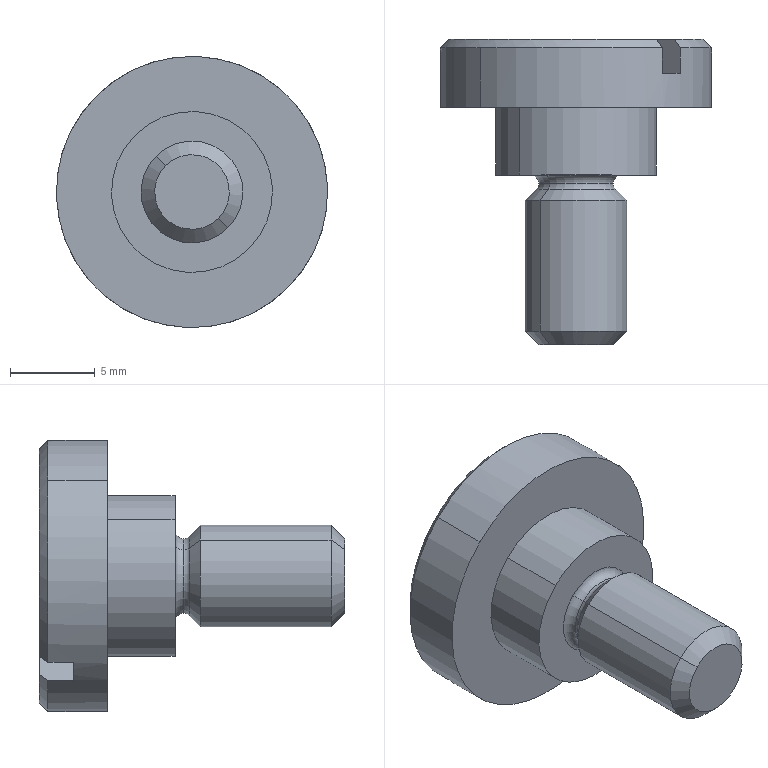Component | SolidWorks | JB_T8045.5-1999DrillBushingScrewM6-1 | 1 solid | 25 faces | box 16 x 18 x 16 mm | volume 1298 mm3 | plane 8 | cone 7 | cylinder 6 | torus 4 | commonest cylinder face diameters 6 x2 9.5 x2 16 x2 | material Nickel
STEP:
#1=COLOUR_RGB('',0.7922,0.8196,0.9333);
#2=FILL_AREA_STYLE_COLOUR('',#1);
#3=FILL_AREA_STYLE('',(#2));
#4=SURFACE_STYLE_FILL_AREA(#3);
#5=SURFACE_SIDE_STYLE('',(#4));
#6=SURFACE_STYLE_USAGE(.BOTH.,#5);
#7=PRESENTATION_STYLE_ASSIGNMENT((#6));
#8=CARTESIAN_POINT('',(0.06125,11.575,1.415));
#9=VERTEX_POINT('',#8);
#10=CARTESIAN_POINT('',(-0.06125,11.575,1.538));
#11=VERTEX_POINT('',#10);
#12=CARTESIAN_POINT('',(0.,11.575,1.476));
#13=DIRECTION('',(0.,-1.,0.));
#14=DIRECTION('',(0.7071,0.,-0.7071));
#15=AXIS2_PLACEMENT_3D('',#12,#13,#14);
#16=CIRCLE('',#15,0.08661);
#17=EDGE_CURVE('',#9,#11,#16,.T.);
#18=ORIENTED_EDGE('',*,*,#17,.F.);
#19=CARTESIAN_POINT('',(0.08352,11.606,1.393));
#20=VERTEX_POINT('',#19);
#21=CARTESIAN_POINT('',(0.06125,11.575,1.415));
#22=DIRECTION('',(0.5,0.7071,-0.5));
#23=VECTOR('',#22,39.37);
#24=LINE('',#21,#23);
#25=EDGE_CURVE('',#9,#20,#24,.T.);
#26=ORIENTED_EDGE('',*,*,#25,.T.);
#27=CARTESIAN_POINT('',(-0.08352,11.606,1.56));
#28=VERTEX_POINT('',#27);
#29=CARTESIAN_POINT('',(0.,11.606,1.476));
#30=DIRECTION('',(0.,1.,0.));
#31=DIRECTION('',(0.7071,0.,-0.7071));
#32=AXIS2_PLACEMENT_3D('',#29,#30,#31);
#33=CIRCLE('',#32,0.1181);
#34=EDGE_CURVE('',#28,#20,#33,.T.);
#35=ORIENTED_EDGE('',*,*,#34,.F.);
#36=CARTESIAN_POINT('',(-0.06125,11.575,1.538));
#37=DIRECTION('',(-0.5,0.7071,0.5));
#38=VECTOR('',#37,39.37);
#39=LINE('',#36,#38);
#40=EDGE_CURVE('',#11,#28,#39,.T.);
#41=ORIENTED_EDGE('',*,*,#40,.F.);
#42=EDGE_LOOP('',(#18,#26,#35,#41));
#43=FACE_OUTER_BOUND('',#42,.T.);
#44=CARTESIAN_POINT('',(0.,11.575,1.476));
#45=DIRECTION('',(0.,1.,0.));
#46=DIRECTION('',(-0.7071,0.,0.7071));
#47=AXIS2_PLACEMENT_3D('',#44,#45,#46);
#48=CONICAL_SURFACE('',#47,0.08661,0.7854);
#49=ADVANCED_FACE('',(#43),#48,.T.);
#50=CARTESIAN_POINT('',(0.06125,11.949,1.415));
#51=VERTEX_POINT('',#50);
#52=CARTESIAN_POINT('',(-0.06125,11.949,1.538));
#53=VERTEX_POINT('',#52);
#54=CARTESIAN_POINT('',(0.,11.949,1.476));
#55=DIRECTION('',(0.,1.,0.));
#56=DIRECTION('',(0.7071,0.,-0.7071));
#57=AXIS2_PLACEMENT_3D('',#54,#55,#56);
#58=CIRCLE('',#57,0.08661);
#59=EDGE_CURVE('',#51,#53,#58,.T.);
#60=ORIENTED_EDGE('',*,*,#59,.T.);
#61=CARTESIAN_POINT('',(-0.07516,11.969,1.552));
#62=VERTEX_POINT('',#61);
#63=CARTESIAN_POINT('',(-0.07516,11.949,1.552));
#64=DIRECTION('',(0.7071,0.,0.7071));
#65=DIRECTION('',(0.7071,0.,-0.7071));
#66=AXIS2_PLACEMENT_3D('',#63,#64,#65);
#67=CIRCLE('',#66,0.01969);
#68=EDGE_CURVE('',#53,#62,#67,.T.);
#69=ORIENTED_EDGE('',*,*,#68,.T.);
#70=CARTESIAN_POINT('',(0.07516,11.969,1.401));
#71=VERTEX_POINT('',#70);
#72=CARTESIAN_POINT('',(0.,11.969,1.476));
#73=DIRECTION('',(0.,1.,0.));
#74=DIRECTION('',(0.7071,0.,-0.7071));
#75=AXIS2_PLACEMENT_3D('',#72,#73,#74);
#76=CIRCLE('',#75,0.1063);
#77=EDGE_CURVE('',#71,#62,#76,.T.);
#78=ORIENTED_EDGE('',*,*,#77,.F.);
#79=CARTESIAN_POINT('',(0.07516,11.949,1.401));
#80=DIRECTION('',(-0.7071,0.,-0.7071));
#81=DIRECTION('',(-0.7071,0.,0.7071));
#82=AXIS2_PLACEMENT_3D('',#79,#80,#81);
#83=CIRCLE('',#82,0.01969);
#84=EDGE_CURVE('',#51,#71,#83,.T.);
#85=ORIENTED_EDGE('',*,*,#84,.F.);
#86=EDGE_LOOP('',(#60,#69,#78,#85));
#87=FACE_OUTER_BOUND('',#86,.T.);
#88=CARTESIAN_POINT('',(0.,11.949,1.476));
#89=DIRECTION('',(0.,-1.,0.));
#90=DIRECTION('',(0.7071,0.,-0.7071));
#91=AXIS2_PLACEMENT_3D('',#88,#89,#90);
#92=TOROIDAL_SURFACE('',#91,0.1063,0.01969);
#93=ADVANCED_FACE('',(#87),#92,.F.);
#94=CARTESIAN_POINT('',(-0.06532,11.935,1.542));
#95=VERTEX_POINT('',#94);
#96=CARTESIAN_POINT('',(0.06532,11.935,1.411));
#97=VERTEX_POINT('',#96);
#98=CARTESIAN_POINT('',(0.,11.935,1.476));
#99=DIRECTION('',(0.,-1.,0.));
#100=DIRECTION('',(-0.7071,0.,0.7071));
#101=AXIS2_PLACEMENT_3D('',#98,#99,#100);
#102=CIRCLE('',#101,0.09238);
#103=EDGE_CURVE('',#95,#97,#102,.T.);
#104=ORIENTED_EDGE('',*,*,#103,.F.);
#105=CARTESIAN_POINT('',(-0.07516,11.949,1.552));
#106=DIRECTION('',(0.7071,0.,0.7071));
#107=DIRECTION('',(0.7071,0.,-0.7071));
#108=AXIS2_PLACEMENT_3D('',#105,#106,#107);
#109=CIRCLE('',#108,0.01969);
#110=EDGE_CURVE('',#95,#53,#109,.T.);
#111=ORIENTED_EDGE('',*,*,#110,.T.);
#112=ORIENTED_EDGE('',*,*,#59,.F.);
#113=CARTESIAN_POINT('',(0.07516,11.949,1.401));
#114=DIRECTION('',(-0.7071,0.,-0.7071));
#115=DIRECTION('',(-0.7071,0.,0.7071));
#116=AXIS2_PLACEMENT_3D('',#113,#114,#115);
#117=CIRCLE('',#116,0.01969);
#118=EDGE_CURVE('',#97,#51,#117,.T.);
#119=ORIENTED_EDGE('',*,*,#118,.F.);
#120=EDGE_LOOP('',(#104,#111,#112,#119));
#121=FACE_OUTER_BOUND('',#120,.T.);
#122=CARTESIAN_POINT('',(0.,11.949,1.476));
#123=DIRECTION('',(0.,-1.,0.));
#124=DIRECTION('',(0.7071,0.,-0.7071));
#125=AXIS2_PLACEMENT_3D('',#122,#123,#124);
#126=TOROIDAL_SURFACE('',#125,0.1063,0.01969);
#127=ADVANCED_FACE('',(#121),#126,.F.);
#128=CARTESIAN_POINT('',(0.,11.935,1.476));
#129=DIRECTION('',(0.,-1.,0.));
#130=DIRECTION('',(-0.7071,0.,0.7071));
#131=AXIS2_PLACEMENT_3D('',#128,#129,#130);
#132=CIRCLE('',#131,0.09238);
#133=EDGE_CURVE('',#97,#95,#132,.T.);
#134=ORIENTED_EDGE('',*,*,#133,.T.);
#135=CARTESIAN_POINT('',(-0.08352,11.909,1.56));
#136=VERTEX_POINT('',#135);
#137=CARTESIAN_POINT('',(-0.08352,11.909,1.56));
#138=DIRECTION('',(-0.5,-0.7071,0.5));
#139=VECTOR('',#138,39.37);
#140=LINE('',#137,#139);
#141=EDGE_CURVE('',#95,#136,#140,.T.);
#142=ORIENTED_EDGE('',*,*,#141,.T.);
#143=CARTESIAN_POINT('',(0.08352,11.909,1.393));
#144=VERTEX_POINT('',#143);
#145=CARTESIAN_POINT('',(0.,11.909,1.476));
#146=DIRECTION('',(0.,-1.,0.));
#147=DIRECTION('',(0.7071,0.,-0.7071));
#148=AXIS2_PLACEMENT_3D('',#145,#146,#147);
#149=CIRCLE('',#148,0.1181);
#150=EDGE_CURVE('',#144,#136,#149,.T.);
#151=ORIENTED_EDGE('',*,*,#150,.F.);
#152=CARTESIAN_POINT('',(0.08352,11.909,1.393));
#153=DIRECTION('',(0.5,-0.7071,-0.5));
#154=VECTOR('',#153,39.37);
#155=LINE('',#152,#154);
#156=EDGE_CURVE('',#97,#144,#155,.T.);
#157=ORIENTED_EDGE('',*,*,#156,.F.);
#158=EDGE_LOOP('',(#134,#142,#151,#157));
#159=FACE_OUTER_BOUND('',#158,.T.);
#160=CARTESIAN_POINT('',(0.,11.909,1.476));
#161=DIRECTION('',(0.,-1.,0.));
#162=DIRECTION('',(0.7071,0.,-0.7071));
#163=AXIS2_PLACEMENT_3D('',#160,#161,#162);
#164=CONICAL_SURFACE('',#163,0.1181,0.7854);
#165=ADVANCED_FACE('',(#159),#164,.T.);
#166=ORIENTED_EDGE('',*,*,#34,.T.);
#167=CARTESIAN_POINT('',(0.08352,11.575,1.393));
#168=DIRECTION('',(0.,1.,0.));
#169=VECTOR('',#168,39.37);
#170=LINE('',#167,#169);
#171=EDGE_CURVE('',#20,#144,#170,.T.);
#172=ORIENTED_EDGE('',*,*,#171,.T.);
#173=ORIENTED_EDGE('',*,*,#150,.T.);
#174=CARTESIAN_POINT('',(-0.08352,11.575,1.56));
#175=DIRECTION('',(0.,1.,0.));
#176=VECTOR('',#175,39.37);
#177=LINE('',#174,#176);
#178=EDGE_CURVE('',#28,#136,#177,.T.);
#179=ORIENTED_EDGE('',*,*,#178,.F.);
#180=EDGE_LOOP('',(#166,#172,#173,#179));
#181=FACE_OUTER_BOUND('',#180,.T.);
#182=CARTESIAN_POINT('',(0.,11.575,1.476));
#183=DIRECTION('',(0.,1.,0.));
#184=DIRECTION('',(-0.7071,0.,0.7071));
#185=AXIS2_PLACEMENT_3D('',#182,#183,#184);
#186=CYLINDRICAL_SURFACE('',#185,0.1181);
#187=ADVANCED_FACE('',(#181),#186,.T.);
#188=CARTESIAN_POINT('',(0.1322,11.969,1.344));
#189=VERTEX_POINT('',#188);
#190=CARTESIAN_POINT('',(-0.1322,11.969,1.609));
#191=VERTEX_POINT('',#190);
#192=CARTESIAN_POINT('',(0.,11.969,1.476));
#193=DIRECTION('',(0.,-1.,0.));
#194=DIRECTION('',(0.7071,0.,-0.7071));
#195=AXIS2_PLACEMENT_3D('',#192,#193,#194);
#196=CIRCLE('',#195,0.187);
#197=EDGE_CURVE('',#189,#191,#196,.T.);
#198=ORIENTED_EDGE('',*,*,#197,.F.);
#199=CARTESIAN_POINT('',(0.1322,12.126,1.344));
#200=VERTEX_POINT('',#199);
#201=CARTESIAN_POINT('',(0.1322,11.969,1.344));
#202=DIRECTION('',(0.,1.,0.));
#203=VECTOR('',#202,39.37);
#204=LINE('',#201,#203);
#205=EDGE_CURVE('',#189,#200,#204,.T.);
#206=ORIENTED_EDGE('',*,*,#205,.T.);
#207=CARTESIAN_POINT('',(-0.1322,12.126,1.609));
#208=VERTEX_POINT('',#207);
#209=CARTESIAN_POINT('',(0.,12.126,1.476));
#210=DIRECTION('',(0.,-1.,0.));
#211=DIRECTION('',(-0.7071,0.,0.7071));
#212=AXIS2_PLACEMENT_3D('',#209,#210,#211);
#213=CIRCLE('',#212,0.187);
#214=EDGE_CURVE('',#200,#208,#213,.T.);
#215=ORIENTED_EDGE('',*,*,#214,.T.);
#216=CARTESIAN_POINT('',(-0.1322,11.969,1.609));
#217=DIRECTION('',(0.,1.,0.));
#218=VECTOR('',#217,39.37);
#219=LINE('',#216,#218);
#220=EDGE_CURVE('',#191,#208,#219,.T.);
#221=ORIENTED_EDGE('',*,*,#220,.F.);
#222=EDGE_LOOP('',(#198,#206,#215,#221));
#223=FACE_OUTER_BOUND('',#222,.T.);
#224=CARTESIAN_POINT('',(0.,11.969,1.476));
#225=DIRECTION('',(0.,1.,0.));
#226=DIRECTION('',(-0.7071,0.,0.7071));
#227=AXIS2_PLACEMENT_3D('',#224,#225,#226);
#228=CYLINDRICAL_SURFACE('',#227,0.187);
#229=ADVANCED_FACE('',(#223),#228,.T.);
#230=CARTESIAN_POINT('',(0.2088,12.283,1.268));
#231=VERTEX_POINT('',#230);
#232=CARTESIAN_POINT('',(-0.1869,12.283,1.248));
#233=VERTEX_POINT('',#232);
#234=CARTESIAN_POINT('',(0.,12.283,1.476));
#235=DIRECTION('',(0.,1.,0.));
#236=DIRECTION('',(-0.7071,0.,0.7071));
#237=AXIS2_PLACEMENT_3D('',#234,#235,#236);
#238=CIRCLE('',#237,0.2953);
#239=EDGE_CURVE('',#231,#233,#238,.T.);
#240=ORIENTED_EDGE('',*,*,#239,.F.);
#241=CARTESIAN_POINT('',(0.2227,12.264,1.254));
#242=VERTEX_POINT('',#241);
#243=CARTESIAN_POINT('',(0.2088,12.283,1.268));
#244=DIRECTION('',(0.5,-0.7071,-0.5));
#245=VECTOR('',#244,39.37);
#246=LINE('',#243,#245);
#247=EDGE_CURVE('',#231,#242,#246,.T.);
#248=ORIENTED_EDGE('',*,*,#247,.T.);
#249=CARTESIAN_POINT('',(-0.2009,12.264,1.234));
#250=VERTEX_POINT('',#249);
#251=CARTESIAN_POINT('',(0.,12.264,1.476));
#252=DIRECTION('',(0.,-1.,0.));
#253=DIRECTION('',(-0.7071,0.,0.7071));
#254=AXIS2_PLACEMENT_3D('',#251,#252,#253);
#255=CIRCLE('',#254,0.315);
#256=EDGE_CURVE('',#250,#242,#255,.T.);
#257=ORIENTED_EDGE('',*,*,#256,.F.);
#258=CARTESIAN_POINT('',(-0.1869,12.283,1.248));
#259=CARTESIAN_POINT('',(-0.1915,12.277,1.243));
#260=CARTESIAN_POINT('',(-0.1962,12.27,1.238));
#261=CARTESIAN_POINT('',(-0.2009,12.264,1.234));
#262=B_SPLINE_CURVE_WITH_KNOTS('',3,(#258,#259,#260,#261),.UNSPECIFIED.,.F.,.F.,(4,4),(0.03463,0.03534),.UNSPECIFIED.);
#263=EDGE_CURVE('',#233,#250,#262,.T.);
#264=ORIENTED_EDGE('',*,*,#263,.F.);
#265=EDGE_LOOP('',(#240,#248,#257,#264));
#266=FACE_OUTER_BOUND('',#265,.T.);
#267=CARTESIAN_POINT('',(0.,12.283,1.476));
#268=DIRECTION('',(0.,-1.,0.));
#269=DIRECTION('',(0.7071,0.,-0.7071));
#270=AXIS2_PLACEMENT_3D('',#267,#268,#269);
#271=CONICAL_SURFACE('',#270,0.2953,0.7854);
#272=ADVANCED_FACE('',(#266),#271,.T.);
#273=CARTESIAN_POINT('',(-0.2227,12.126,1.699));
#274=VERTEX_POINT('',#273);
#275=CARTESIAN_POINT('',(0.2227,12.126,1.254));
#276=VERTEX_POINT('',#275);
#277=CARTESIAN_POINT('',(0.,12.126,1.476));
#278=DIRECTION('',(0.,1.,0.));
#279=DIRECTION('',(-0.7071,0.,0.7071));
#280=AXIS2_PLACEMENT_3D('',#277,#278,#279);
#281=CIRCLE('',#280,0.315);
#282=EDGE_CURVE('',#274,#276,#281,.T.);
#283=ORIENTED_EDGE('',*,*,#282,.T.);
#284=CARTESIAN_POINT('',(0.2227,12.126,1.254));
#285=DIRECTION('',(0.,1.,0.));
#286=VECTOR('',#285,39.37);
#287=LINE('',#284,#286);
#288=EDGE_CURVE('',#276,#242,#287,.T.);
#289=ORIENTED_EDGE('',*,*,#288,.T.);
#290=CARTESIAN_POINT('',(0.2426,12.264,1.677));
#291=VERTEX_POINT('',#290);
#292=CARTESIAN_POINT('',(0.,12.264,1.476));
#293=DIRECTION('',(0.,-1.,0.));
#294=DIRECTION('',(-0.7071,0.,0.7071));
#295=AXIS2_PLACEMENT_3D('',#292,#293,#294);
#296=CIRCLE('',#295,0.315);
#297=EDGE_CURVE('',#242,#291,#296,.T.);
#298=ORIENTED_EDGE('',*,*,#297,.T.);
#299=CARTESIAN_POINT('',(0.2426,12.205,1.677));
#300=VERTEX_POINT('',#299);
#301=CARTESIAN_POINT('',(0.2426,12.126,1.677));
#302=DIRECTION('',(0.,1.,0.));
#303=VECTOR('',#302,39.37);
#304=LINE('',#301,#303);
#305=EDGE_CURVE('',#300,#291,#304,.T.);
#306=ORIENTED_EDGE('',*,*,#305,.F.);
#307=CARTESIAN_POINT('',(0.2009,12.205,1.719));
#308=VERTEX_POINT('',#307);
#309=CARTESIAN_POINT('',(0.,12.205,1.476));
#310=DIRECTION('',(0.,1.,0.));
#311=DIRECTION('',(0.7071,0.,-0.7071));
#312=AXIS2_PLACEMENT_3D('',#309,#310,#311);
#313=CIRCLE('',#312,0.315);
#314=EDGE_CURVE('',#308,#300,#313,.T.);
#315=ORIENTED_EDGE('',*,*,#314,.F.);
#316=CARTESIAN_POINT('',(0.2009,12.264,1.719));
#317=VERTEX_POINT('',#316);
#318=CARTESIAN_POINT('',(0.2009,12.126,1.719));
#319=DIRECTION('',(0.,-1.,0.));
#320=VECTOR('',#319,39.37);
#321=LINE('',#318,#320);
#322=EDGE_CURVE('',#317,#308,#321,.T.);
#323=ORIENTED_EDGE('',*,*,#322,.F.);
#324=CARTESIAN_POINT('',(-0.2227,12.264,1.699));
#325=VERTEX_POINT('',#324);
#326=CARTESIAN_POINT('',(0.,12.264,1.476));
#327=DIRECTION('',(0.,-1.,0.));
#328=DIRECTION('',(-0.7071,0.,0.7071));
#329=AXIS2_PLACEMENT_3D('',#326,#327,#328);
#330=CIRCLE('',#329,0.315);
#331=EDGE_CURVE('',#317,#325,#330,.T.);
#332=ORIENTED_EDGE('',*,*,#331,.T.);
#333=CARTESIAN_POINT('',(-0.2227,12.126,1.699));
#334=DIRECTION('',(0.,1.,0.));
#335=VECTOR('',#334,39.37);
#336=LINE('',#333,#335);
#337=EDGE_CURVE('',#274,#325,#336,.T.);
#338=ORIENTED_EDGE('',*,*,#337,.F.);
#339=EDGE_LOOP('',(#283,#289,#298,#306,#315,#323,#332,#338));
#340=FACE_OUTER_BOUND('',#339,.T.);
#341=CARTESIAN_POINT('',(0.,12.126,1.476));
#342=DIRECTION('',(0.,1.,0.));
#343=DIRECTION('',(-0.7071,0.,0.7071));
#344=AXIS2_PLACEMENT_3D('',#341,#342,#343);
#345=CYLINDRICAL_SURFACE('',#344,0.315);
#346=ADVANCED_FACE('',(#340),#345,.T.);
#347=ORIENTED_EDGE('',*,*,#77,.T.);
#348=CARTESIAN_POINT('',(0.,11.969,1.476));
#349=DIRECTION('',(0.,1.,0.));
#350=DIRECTION('',(0.7071,0.,-0.7071));
#351=AXIS2_PLACEMENT_3D('',#348,#349,#350);
#352=CIRCLE('',#351,0.1063);
#353=EDGE_CURVE('',#62,#71,#352,.T.);
#354=ORIENTED_EDGE('',*,*,#353,.T.);
#355=EDGE_LOOP('',(#347,#354));
#356=FACE_BOUND('',#355,.T.);
#357=CARTESIAN_POINT('',(0.,11.969,1.476));
#358=DIRECTION('',(0.,-1.,0.));
#359=DIRECTION('',(0.7071,0.,-0.7071));
#360=AXIS2_PLACEMENT_3D('',#357,#358,#359);
#361=CIRCLE('',#360,0.187);
#362=EDGE_CURVE('',#191,#189,#361,.T.);
#363=ORIENTED_EDGE('',*,*,#362,.T.);
#364=ORIENTED_EDGE('',*,*,#197,.T.);
#365=EDGE_LOOP('',(#363,#364));
#366=FACE_OUTER_BOUND('',#365,.T.);
#367=CARTESIAN_POINT('',(0.,11.969,1.476));
#368=DIRECTION('',(0.,-1.,0.));
#369=DIRECTION('',(0.7071,0.,-0.7071));
#370=AXIS2_PLACEMENT_3D('',#367,#368,#369);
#371=PLANE('',#370);
#372=ADVANCED_FACE('',(#356,#366),#371,.T.);
#373=ORIENTED_EDGE('',*,*,#282,.F.);
#374=CARTESIAN_POINT('',(0.,12.126,1.476));
#375=DIRECTION('',(0.,1.,0.));
#376=DIRECTION('',(-0.7071,0.,0.7071));
#377=AXIS2_PLACEMENT_3D('',#374,#375,#376);
#378=CIRCLE('',#377,0.315);
#379=EDGE_CURVE('',#276,#274,#378,.T.);
#380=ORIENTED_EDGE('',*,*,#379,.F.);
#381=EDGE_LOOP('',(#373,#380));
#382=FACE_OUTER_BOUND('',#381,.T.);
#383=CARTESIAN_POINT('',(0.,12.126,1.476));
#384=DIRECTION('',(0.,-1.,0.));
#385=DIRECTION('',(-0.7071,0.,0.7071));
#386=AXIS2_PLACEMENT_3D('',#383,#384,#385);
#387=CIRCLE('',#386,0.187);
#388=EDGE_CURVE('',#208,#200,#387,.T.);
#389=ORIENTED_EDGE('',*,*,#388,.F.);
#390=ORIENTED_EDGE('',*,*,#214,.F.);
#391=EDGE_LOOP('',(#389,#390));
#392=FACE_BOUND('',#391,.T.);
#393=CARTESIAN_POINT('',(0.,12.126,1.476));
#394=DIRECTION('',(0.,1.,0.));
#395=DIRECTION('',(-0.7071,0.,0.7071));
#396=AXIS2_PLACEMENT_3D('',#393,#394,#395);
#397=PLANE('',#396);
#398=ADVANCED_FACE('',(#382,#392),#397,.F.);
#399=CARTESIAN_POINT('',(-0.2286,12.283,1.29));
#400=VERTEX_POINT('',#399);
#401=CARTESIAN_POINT('',(0.1869,12.283,1.705));
#402=VERTEX_POINT('',#401);
#403=CARTESIAN_POINT('',(0.706,12.283,2.224));
#404=DIRECTION('',(0.7071,0.,0.7071));
#405=VECTOR('',#404,39.37);
#406=LINE('',#403,#405);
#407=EDGE_CURVE('',#400,#402,#406,.T.);
#408=ORIENTED_EDGE('',*,*,#407,.F.);
#409=CARTESIAN_POINT('',(0.,12.283,1.476));
#410=DIRECTION('',(0.,1.,0.));
#411=DIRECTION('',(-0.7071,0.,0.7071));
#412=AXIS2_PLACEMENT_3D('',#409,#410,#411);
#413=CIRCLE('',#412,0.2953);
#414=EDGE_CURVE('',#400,#402,#413,.T.);
#415=ORIENTED_EDGE('',*,*,#414,.T.);
#416=EDGE_LOOP('',(#408,#415));
#417=FACE_OUTER_BOUND('',#416,.T.);
#418=CARTESIAN_POINT('',(0.,12.283,1.476));
#419=DIRECTION('',(0.,1.,0.));
#420=DIRECTION('',(-0.7071,0.,0.7071));
#421=AXIS2_PLACEMENT_3D('',#418,#419,#420);
#422=PLANE('',#421);
#423=ADVANCED_FACE('',(#417),#422,.T.);
#424=CARTESIAN_POINT('',(-0.2426,12.264,1.276));
#425=VERTEX_POINT('',#424);
#426=CARTESIAN_POINT('',(-0.2426,12.264,1.276));
#427=CARTESIAN_POINT('',(-0.2379,12.27,1.28));
#428=CARTESIAN_POINT('',(-0.2333,12.277,1.285));
#429=CARTESIAN_POINT('',(-0.2286,12.283,1.29));
#430=B_SPLINE_CURVE_WITH_KNOTS('',3,(#426,#427,#428,#429),.UNSPECIFIED.,.F.,.F.,(4,4),(0.0136,0.01431),.UNSPECIFIED.);
#431=EDGE_CURVE('',#425,#400,#430,.T.);
#432=ORIENTED_EDGE('',*,*,#431,.F.);
#433=CARTESIAN_POINT('',(0.,12.264,1.476));
#434=DIRECTION('',(0.,-1.,0.));
#435=DIRECTION('',(-0.7071,0.,0.7071));
#436=AXIS2_PLACEMENT_3D('',#433,#434,#435);
#437=CIRCLE('',#436,0.315);
#438=EDGE_CURVE('',#325,#425,#437,.T.);
#439=ORIENTED_EDGE('',*,*,#438,.F.);
#440=ORIENTED_EDGE('',*,*,#331,.F.);
#441=CARTESIAN_POINT('',(0.1869,12.283,1.705));
#442=CARTESIAN_POINT('',(0.1915,12.277,1.71));
#443=CARTESIAN_POINT('',(0.1962,12.27,1.714));
#444=CARTESIAN_POINT('',(0.2009,12.264,1.719));
#445=B_SPLINE_CURVE_WITH_KNOTS('',3,(#441,#442,#443,#444),.UNSPECIFIED.,.F.,.F.,(4,4),(0.03463,0.03534),.UNSPECIFIED.);
#446=EDGE_CURVE('',#402,#317,#445,.T.);
#447=ORIENTED_EDGE('',*,*,#446,.F.);
#448=ORIENTED_EDGE('',*,*,#414,.F.);
#449=EDGE_LOOP('',(#432,#439,#440,#447,#448));
#450=FACE_OUTER_BOUND('',#449,.T.);
#451=CARTESIAN_POINT('',(0.,12.283,1.476));
#452=DIRECTION('',(0.,-1.,0.));
#453=DIRECTION('',(0.7071,0.,-0.7071));
#454=AXIS2_PLACEMENT_3D('',#451,#452,#453);
#455=CONICAL_SURFACE('',#454,0.2953,0.7854);
#456=ADVANCED_FACE('',(#450),#455,.T.);
#457=ORIENTED_EDGE('',*,*,#288,.F.);
#458=ORIENTED_EDGE('',*,*,#379,.T.);
#459=ORIENTED_EDGE('',*,*,#337,.T.);
#460=ORIENTED_EDGE('',*,*,#438,.T.);
#461=CARTESIAN_POINT('',(-0.2426,12.205,1.276));
#462=VERTEX_POINT('',#461);
#463=CARTESIAN_POINT('',(-0.2426,12.126,1.276));
#464=DIRECTION('',(0.,1.,0.));
#465=VECTOR('',#464,39.37);
#466=LINE('',#463,#465);
#467=EDGE_CURVE('',#462,#425,#466,.T.);
#468=ORIENTED_EDGE('',*,*,#467,.F.);
#469=CARTESIAN_POINT('',(-0.2009,12.205,1.234));
#470=VERTEX_POINT('',#469);
#471=CARTESIAN_POINT('',(0.,12.205,1.476));
#472=DIRECTION('',(0.,1.,0.));
#473=DIRECTION('',(0.7071,0.,-0.7071));
#474=AXIS2_PLACEMENT_3D('',#471,#472,#473);
#475=CIRCLE('',#474,0.315);
#476=EDGE_CURVE('',#470,#462,#475,.T.);
#477=ORIENTED_EDGE('',*,*,#476,.F.);
#478=CARTESIAN_POINT('',(-0.2009,12.126,1.234));
#479=DIRECTION('',(0.,-1.,0.));
#480=VECTOR('',#479,39.37);
#481=LINE('',#478,#480);
#482=EDGE_CURVE('',#250,#470,#481,.T.);
#483=ORIENTED_EDGE('',*,*,#482,.F.);
#484=ORIENTED_EDGE('',*,*,#256,.T.);
#485=EDGE_LOOP('',(#457,#458,#459,#460,#468,#477,#483,#484));
#486=FACE_OUTER_BOUND('',#485,.T.);
#487=CARTESIAN_POINT('',(0.,12.126,1.476));
#488=DIRECTION('',(0.,1.,0.));
#489=DIRECTION('',(-0.7071,0.,0.7071));
#490=AXIS2_PLACEMENT_3D('',#487,#488,#489);
#491=CYLINDRICAL_SURFACE('',#490,0.315);
#492=ADVANCED_FACE('',(#486),#491,.T.);
#493=CARTESIAN_POINT('',(0.2286,12.283,1.663));
#494=VERTEX_POINT('',#493);
#495=CARTESIAN_POINT('',(0.7477,12.283,2.182));
#496=DIRECTION('',(-0.7071,0.,-0.7071));
#497=VECTOR('',#496,39.37);
#498=LINE('',#495,#497);
#499=EDGE_CURVE('',#494,#233,#498,.T.);
#500=ORIENTED_EDGE('',*,*,#499,.F.);
#501=CARTESIAN_POINT('',(0.,12.283,1.476));
#502=DIRECTION('',(0.,1.,0.));
#503=DIRECTION('',(-0.7071,0.,0.7071));
#504=AXIS2_PLACEMENT_3D('',#501,#502,#503);
#505=CIRCLE('',#504,0.2953);
#506=EDGE_CURVE('',#494,#231,#505,.T.);
#507=ORIENTED_EDGE('',*,*,#506,.T.);
#508=ORIENTED_EDGE('',*,*,#239,.T.);
#509=EDGE_LOOP('',(#500,#507,#508));
#510=FACE_OUTER_BOUND('',#509,.T.);
#511=CARTESIAN_POINT('',(0.,12.283,1.476));
#512=DIRECTION('',(0.,1.,0.));
#513=DIRECTION('',(-0.7071,0.,0.7071));
#514=AXIS2_PLACEMENT_3D('',#511,#512,#513);
#515=PLANE('',#514);
#516=ADVANCED_FACE('',(#510),#515,.T.);
#517=ORIENTED_EDGE('',*,*,#247,.F.);
#518=ORIENTED_EDGE('',*,*,#506,.F.);
#519=CARTESIAN_POINT('',(0.2426,12.264,1.677));
#520=CARTESIAN_POINT('',(0.2379,12.27,1.673));
#521=CARTESIAN_POINT('',(0.2333,12.277,1.668));
#522=CARTESIAN_POINT('',(0.2286,12.283,1.663));
#523=B_SPLINE_CURVE_WITH_KNOTS('',3,(#519,#520,#521,#522),.UNSPECIFIED.,.F.,.F.,(4,4),(0.0136,0.01431),.UNSPECIFIED.);
#524=EDGE_CURVE('',#291,#494,#523,.T.);
#525=ORIENTED_EDGE('',*,*,#524,.F.);
#526=ORIENTED_EDGE('',*,*,#297,.F.);
#527=EDGE_LOOP('',(#517,#518,#525,#526));
#528=FACE_OUTER_BOUND('',#527,.T.);
#529=CARTESIAN_POINT('',(0.,12.283,1.476));
#530=DIRECTION('',(0.,-1.,0.));
#531=DIRECTION('',(0.7071,0.,-0.7071));
#532=AXIS2_PLACEMENT_3D('',#529,#530,#531);
#533=CONICAL_SURFACE('',#532,0.2953,0.7854);
#534=ADVANCED_FACE('',(#528),#533,.T.);
#535=ORIENTED_EDGE('',*,*,#467,.T.);
#536=ORIENTED_EDGE('',*,*,#431,.T.);
#537=ORIENTED_EDGE('',*,*,#407,.T.);
#538=ORIENTED_EDGE('',*,*,#446,.T.);
#539=ORIENTED_EDGE('',*,*,#322,.T.);
#540=CARTESIAN_POINT('',(0.706,12.205,2.224));
#541=DIRECTION('',(0.7071,0.,0.7071));
#542=VECTOR('',#541,39.37);
#543=LINE('',#540,#542);
#544=EDGE_CURVE('',#462,#308,#543,.T.);
#545=ORIENTED_EDGE('',*,*,#544,.F.);
#546=EDGE_LOOP('',(#535,#536,#537,#538,#539,#545));
#547=FACE_OUTER_BOUND('',#546,.T.);
#548=CARTESIAN_POINT('',(0.706,12.205,2.224));
#549=DIRECTION('',(-0.7071,0.,0.7071));
#550=DIRECTION('',(0.7071,0.,0.7071));
#551=AXIS2_PLACEMENT_3D('',#548,#549,#550);
#552=PLANE('',#551);
#553=ADVANCED_FACE('',(#547),#552,.F.);
#554=ORIENTED_EDGE('',*,*,#305,.T.);
#555=ORIENTED_EDGE('',*,*,#524,.T.);
#556=ORIENTED_EDGE('',*,*,#499,.T.);
#557=ORIENTED_EDGE('',*,*,#263,.T.);
#558=ORIENTED_EDGE('',*,*,#482,.T.);
#559=CARTESIAN_POINT('',(0.7477,12.205,2.182));
#560=DIRECTION('',(-0.7071,0.,-0.7071));
#561=VECTOR('',#560,39.37);
#562=LINE('',#559,#561);
#563=EDGE_CURVE('',#300,#470,#562,.T.);
#564=ORIENTED_EDGE('',*,*,#563,.F.);
#565=EDGE_LOOP('',(#554,#555,#556,#557,#558,#564));
#566=FACE_OUTER_BOUND('',#565,.T.);
#567=CARTESIAN_POINT('',(0.7477,12.205,2.182));
#568=DIRECTION('',(0.7071,0.,-0.7071));
#569=DIRECTION('',(-0.7071,0.,-0.7071));
#570=AXIS2_PLACEMENT_3D('',#567,#568,#569);
#571=PLANE('',#570);
#572=ADVANCED_FACE('',(#566),#571,.F.);
#573=ORIENTED_EDGE('',*,*,#476,.T.);
#574=ORIENTED_EDGE('',*,*,#544,.T.);
#575=ORIENTED_EDGE('',*,*,#314,.T.);
#576=ORIENTED_EDGE('',*,*,#563,.T.);
#577=EDGE_LOOP('',(#573,#574,#575,#576));
#578=FACE_OUTER_BOUND('',#577,.T.);
#579=CARTESIAN_POINT('',(0.7477,12.205,2.182));
#580=DIRECTION('',(0.,-1.,0.));
#581=DIRECTION('',(0.7071,0.,-0.7071));
#582=AXIS2_PLACEMENT_3D('',#579,#580,#581);
#583=PLANE('',#582);
#584=ADVANCED_FACE('',(#578),#583,.F.);
#585=ORIENTED_EDGE('',*,*,#205,.F.);
#586=ORIENTED_EDGE('',*,*,#362,.F.);
#587=ORIENTED_EDGE('',*,*,#220,.T.);
#588=ORIENTED_EDGE('',*,*,#388,.T.);
#589=EDGE_LOOP('',(#585,#586,#587,#588));
#590=FACE_OUTER_BOUND('',#589,.T.);
#591=CARTESIAN_POINT('',(0.,11.969,1.476));
#592=DIRECTION('',(0.,1.,0.));
#593=DIRECTION('',(-0.7071,0.,0.7071));
#594=AXIS2_PLACEMENT_3D('',#591,#592,#593);
#595=CYLINDRICAL_SURFACE('',#594,0.187);
#596=ADVANCED_FACE('',(#590),#595,.T.);
#597=ORIENTED_EDGE('',*,*,#171,.F.);
#598=CARTESIAN_POINT('',(0.,11.606,1.476));
#599=DIRECTION('',(0.,1.,0.));
#600=DIRECTION('',(0.7071,0.,-0.7071));
#601=AXIS2_PLACEMENT_3D('',#598,#599,#600);
#602=CIRCLE('',#601,0.1181);
#603=EDGE_CURVE('',#20,#28,#602,.T.);
#604=ORIENTED_EDGE('',*,*,#603,.T.);
#605=ORIENTED_EDGE('',*,*,#178,.T.);
#606=CARTESIAN_POINT('',(0.,11.909,1.476));
#607=DIRECTION('',(0.,-1.,0.));
#608=DIRECTION('',(0.7071,0.,-0.7071));
#609=AXIS2_PLACEMENT_3D('',#606,#607,#608);
#610=CIRCLE('',#609,0.1181);
#611=EDGE_CURVE('',#136,#144,#610,.T.);
#612=ORIENTED_EDGE('',*,*,#611,.T.);
#613=EDGE_LOOP('',(#597,#604,#605,#612));
#614=FACE_OUTER_BOUND('',#613,.T.);
#615=CARTESIAN_POINT('',(0.,11.575,1.476));
#616=DIRECTION('',(0.,1.,0.));
#617=DIRECTION('',(-0.7071,0.,0.7071));
#618=AXIS2_PLACEMENT_3D('',#615,#616,#617);
#619=CYLINDRICAL_SURFACE('',#618,0.1181);
#620=ADVANCED_FACE('',(#614),#619,.T.);
#621=CARTESIAN_POINT('',(0.,11.575,1.476));
#622=DIRECTION('',(0.,-1.,0.));
#623=DIRECTION('',(0.7071,0.,-0.7071));
#624=AXIS2_PLACEMENT_3D('',#621,#622,#623);
#625=CIRCLE('',#624,0.08661);
#626=EDGE_CURVE('',#11,#9,#625,.T.);
#627=ORIENTED_EDGE('',*,*,#626,.T.);
#628=ORIENTED_EDGE('',*,*,#17,.T.);
#629=EDGE_LOOP('',(#627,#628));
#630=FACE_OUTER_BOUND('',#629,.T.);
#631=CARTESIAN_POINT('',(0.,11.575,1.476));
#632=DIRECTION('',(0.,-1.,0.));
#633=DIRECTION('',(0.7071,0.,-0.7071));
#634=AXIS2_PLACEMENT_3D('',#631,#632,#633);
#635=PLANE('',#634);
#636=ADVANCED_FACE('',(#630),#635,.T.);
#637=ORIENTED_EDGE('',*,*,#141,.F.);
#638=ORIENTED_EDGE('',*,*,#103,.T.);
#639=ORIENTED_EDGE('',*,*,#156,.T.);
#640=ORIENTED_EDGE('',*,*,#611,.F.);
#641=EDGE_LOOP('',(#637,#638,#639,#640));
#642=FACE_OUTER_BOUND('',#641,.T.);
#643=CARTESIAN_POINT('',(0.,11.909,1.476));
#644=DIRECTION('',(0.,-1.,0.));
#645=DIRECTION('',(0.7071,0.,-0.7071));
#646=AXIS2_PLACEMENT_3D('',#643,#644,#645);
#647=CONICAL_SURFACE('',#646,0.1181,0.7854);
#648=ADVANCED_FACE('',(#642),#647,.T.);
#649=ORIENTED_EDGE('',*,*,#110,.F.);
#650=ORIENTED_EDGE('',*,*,#133,.F.);
#651=ORIENTED_EDGE('',*,*,#118,.T.);
#652=CARTESIAN_POINT('',(0.,11.949,1.476));
#653=DIRECTION('',(0.,1.,0.));
#654=DIRECTION('',(0.7071,0.,-0.7071));
#655=AXIS2_PLACEMENT_3D('',#652,#653,#654);
#656=CIRCLE('',#655,0.08661);
#657=EDGE_CURVE('',#53,#51,#656,.T.);
#658=ORIENTED_EDGE('',*,*,#657,.F.);
#659=EDGE_LOOP('',(#649,#650,#651,#658));
#660=FACE_OUTER_BOUND('',#659,.T.);
#661=CARTESIAN_POINT('',(0.,11.949,1.476));
#662=DIRECTION('',(0.,-1.,0.));
#663=DIRECTION('',(0.7071,0.,-0.7071));
#664=AXIS2_PLACEMENT_3D('',#661,#662,#663);
#665=TOROIDAL_SURFACE('',#664,0.1063,0.01969);
#666=ADVANCED_FACE('',(#660),#665,.F.);
#667=ORIENTED_EDGE('',*,*,#68,.F.);
#668=ORIENTED_EDGE('',*,*,#657,.T.);
#669=ORIENTED_EDGE('',*,*,#84,.T.);
#670=ORIENTED_EDGE('',*,*,#353,.F.);
#671=EDGE_LOOP('',(#667,#668,#669,#670));
#672=FACE_OUTER_BOUND('',#671,.T.);
#673=CARTESIAN_POINT('',(0.,11.949,1.476));
#674=DIRECTION('',(0.,-1.,0.));
#675=DIRECTION('',(0.7071,0.,-0.7071));
#676=AXIS2_PLACEMENT_3D('',#673,#674,#675);
#677=TOROIDAL_SURFACE('',#676,0.1063,0.01969);
#678=ADVANCED_FACE('',(#672),#677,.F.);
#679=ORIENTED_EDGE('',*,*,#25,.F.);
#680=ORIENTED_EDGE('',*,*,#626,.F.);
#681=ORIENTED_EDGE('',*,*,#40,.T.);
#682=ORIENTED_EDGE('',*,*,#603,.F.);
#683=EDGE_LOOP('',(#679,#680,#681,#682));
#684=FACE_OUTER_BOUND('',#683,.T.);
#685=CARTESIAN_POINT('',(0.,11.575,1.476));
#686=DIRECTION('',(0.,1.,0.));
#687=DIRECTION('',(-0.7071,0.,0.7071));
#688=AXIS2_PLACEMENT_3D('',#685,#686,#687);
#689=CONICAL_SURFACE('',#688,0.08661,0.7854);
#690=ADVANCED_FACE('',(#684),#689,.T.);
#691=CLOSED_SHELL('',(#49,#93,#127,#165,#187,#229,#272,#346,#372,#398,#423,#456,#492,#516,#534,#553,#572,#584,#596,#620,#636,#648,#666,#678,#690));
#692=MANIFOLD_SOLID_BREP('',#691);
#693=STYLED_ITEM('',(#7),#692);
#694=PRESENTATION_LAYER_ASSIGNMENT('','',(#693));
#695=CARTESIAN_POINT('',(0.,0.,0.));
#696=DIRECTION('',(0.,0.,1.));
#697=DIRECTION('',(1.,0.,0.));
#698=AXIS2_PLACEMENT_3D('',#695,#696,#697);
#699=(LENGTH_UNIT()NAMED_UNIT(*)SI_UNIT($,.METRE.));
#700=LENGTH_MEASURE_WITH_UNIT(LENGTH_MEASURE(0.0254),#699);
#701=DIMENSIONAL_EXPONENTS(1.,0.,0.,0.,0.,0.,0.);
#702=(CONVERSION_BASED_UNIT('',#700)LENGTH_UNIT()NAMED_UNIT(#701));
#703=UNCERTAINTY_MEASURE_WITH_UNIT(LENGTH_MEASURE(0.00001),#702,'','');
#704=(NAMED_UNIT(*)PLANE_ANGLE_UNIT()SI_UNIT($,.RADIAN.));
#705=(NAMED_UNIT(*)SI_UNIT($,.STERADIAN.)SOLID_ANGLE_UNIT());
#706=(GEOMETRIC_REPRESENTATION_CONTEXT(3)GLOBAL_UNCERTAINTY_ASSIGNED_CONTEXT((#703))GLOBAL_UNIT_ASSIGNED_CONTEXT((#702,#704,#705))REPRESENTATION_CONTEXT('',''));
#707=ADVANCED_BREP_SHAPE_REPRESENTATION('',(#692,#698),#706);
#708=(LENGTH_UNIT()NAMED_UNIT(*)SI_UNIT($,.METRE.));
#709=LENGTH_MEASURE_WITH_UNIT(LENGTH_MEASURE(0.0254),#708);
#710=DIMENSIONAL_EXPONENTS(1.,0.,0.,0.,0.,0.,0.);
#711=(CONVERSION_BASED_UNIT('',#709)LENGTH_UNIT()NAMED_UNIT(#710));
#712=UNCERTAINTY_MEASURE_WITH_UNIT(LENGTH_MEASURE(0.00001),#711,'','');
#713=(NAMED_UNIT(*)PLANE_ANGLE_UNIT()SI_UNIT($,.RADIAN.));
#714=(NAMED_UNIT(*)SI_UNIT($,.STERADIAN.)SOLID_ANGLE_UNIT());
#715=(GEOMETRIC_REPRESENTATION_CONTEXT(3)GLOBAL_UNCERTAINTY_ASSIGNED_CONTEXT((#712))GLOBAL_UNIT_ASSIGNED_CONTEXT((#711,#713,#714))REPRESENTATION_CONTEXT('',''));
#716=MECHANICAL_DESIGN_GEOMETRIC_PRESENTATION_REPRESENTATION('',(#693),#715);